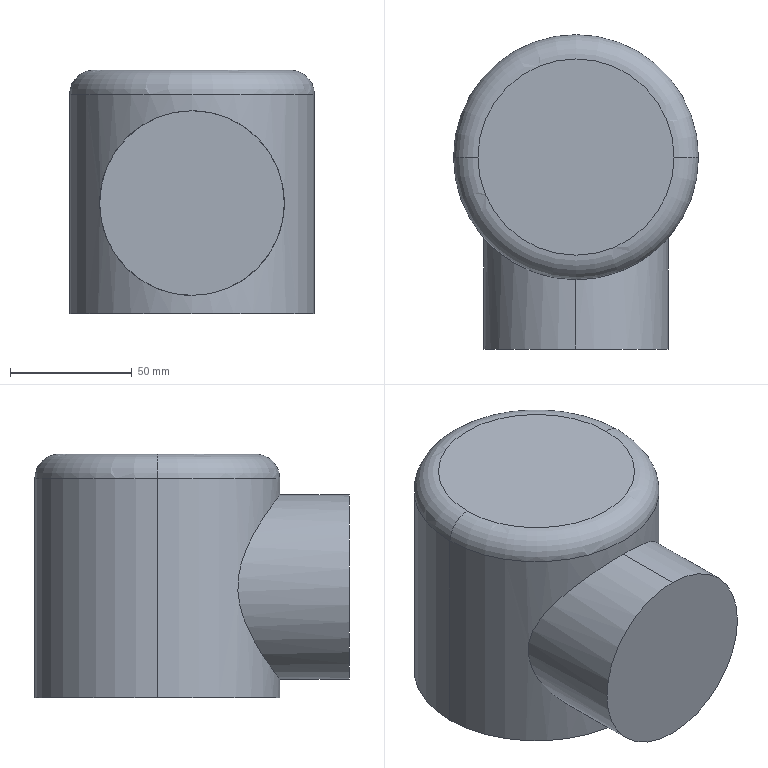Component | SolidWorks | RehabilitationChair-18-3-2 | 1 solid | 9 faces | box 100.49 x 128.95 x 100 mm | volume 932353 mm3 | cylinder 4 | plane 3 | torus 2 | commonest cylinder face diameters 75.746 x2 100.487 x2
STEP:
#1=COLOUR_RGB('',0.7922,0.8196,0.9333);
#2=FILL_AREA_STYLE_COLOUR('',#1);
#3=FILL_AREA_STYLE('',(#2));
#4=SURFACE_STYLE_FILL_AREA(#3);
#5=SURFACE_SIDE_STYLE('',(#4));
#6=SURFACE_STYLE_USAGE(.BOTH.,#5);
#7=PRESENTATION_STYLE_ASSIGNMENT((#6));
#8=CARTESIAN_POINT('',(-6.121,17.859,6.194));
#9=VERTEX_POINT('',#8);
#10=CARTESIAN_POINT('',(-6.121,17.859,3.212));
#11=VERTEX_POINT('',#10);
#12=CARTESIAN_POINT('',(-6.121,17.859,6.194));
#13=CARTESIAN_POINT('',(-6.224,17.859,6.194));
#14=CARTESIAN_POINT('',(-6.325,17.867,6.184));
#15=CARTESIAN_POINT('',(-6.449,17.886,6.158));
#16=CARTESIAN_POINT('',(-6.473,17.89,6.152));
#17=CARTESIAN_POINT('',(-6.522,17.9,6.139));
#18=CARTESIAN_POINT('',(-6.547,17.905,6.132));
#19=CARTESIAN_POINT('',(-6.619,17.922,6.11));
#20=CARTESIAN_POINT('',(-6.665,17.935,6.092));
#21=CARTESIAN_POINT('',(-6.755,17.963,6.053));
#22=CARTESIAN_POINT('',(-6.799,17.978,6.032));
#23=CARTESIAN_POINT('',(-6.863,18.003,5.997));
#24=CARTESIAN_POINT('',(-6.884,18.012,5.985));
#25=CARTESIAN_POINT('',(-6.925,18.029,5.959));
#26=CARTESIAN_POINT('',(-6.945,18.039,5.946));
#27=CARTESIAN_POINT('',(-7.044,18.085,5.878));
#28=CARTESIAN_POINT('',(-7.116,18.125,5.818));
#29=CARTESIAN_POINT('',(-7.198,18.178,5.735));
#30=CARTESIAN_POINT('',(-7.214,18.188,5.718));
#31=CARTESIAN_POINT('',(-7.245,18.209,5.683));
#32=CARTESIAN_POINT('',(-7.261,18.22,5.665));
#33=CARTESIAN_POINT('',(-7.305,18.252,5.611));
#34=CARTESIAN_POINT('',(-7.333,18.273,5.573));
#35=CARTESIAN_POINT('',(-7.41,18.336,5.457));
#36=CARTESIAN_POINT('',(-7.455,18.376,5.375));
#37=CARTESIAN_POINT('',(-7.512,18.43,5.243));
#38=CARTESIAN_POINT('',(-7.529,18.447,5.197));
#39=CARTESIAN_POINT('',(-7.558,18.478,5.103));
#40=CARTESIAN_POINT('',(-7.571,18.491,5.055));
#41=CARTESIAN_POINT('',(-7.586,18.508,4.982));
#42=CARTESIAN_POINT('',(-7.59,18.513,4.957));
#43=CARTESIAN_POINT('',(-7.598,18.521,4.907));
#44=CARTESIAN_POINT('',(-7.601,18.525,4.882));
#45=CARTESIAN_POINT('',(-7.609,18.534,4.805));
#46=CARTESIAN_POINT('',(-7.612,18.537,4.754));
#47=CARTESIAN_POINT('',(-7.612,18.537,4.652));
#48=CARTESIAN_POINT('',(-7.609,18.534,4.601));
#49=CARTESIAN_POINT('',(-7.601,18.525,4.525));
#50=CARTESIAN_POINT('',(-7.598,18.522,4.5));
#51=CARTESIAN_POINT('',(-7.59,18.513,4.45));
#52=CARTESIAN_POINT('',(-7.586,18.508,4.425));
#53=CARTESIAN_POINT('',(-7.571,18.491,4.351));
#54=CARTESIAN_POINT('',(-7.558,18.478,4.303));
#55=CARTESIAN_POINT('',(-7.529,18.447,4.209));
#56=CARTESIAN_POINT('',(-7.512,18.43,4.164));
#57=CARTESIAN_POINT('',(-7.455,18.376,4.031));
#58=CARTESIAN_POINT('',(-7.41,18.335,3.949));
#59=CARTESIAN_POINT('',(-7.332,18.273,3.833));
#60=CARTESIAN_POINT('',(-7.304,18.252,3.795));
#61=CARTESIAN_POINT('',(-7.26,18.22,3.741));
#62=CARTESIAN_POINT('',(-7.244,18.209,3.723));
#63=CARTESIAN_POINT('',(-7.213,18.188,3.688));
#64=CARTESIAN_POINT('',(-7.197,18.177,3.671));
#65=CARTESIAN_POINT('',(-7.115,18.125,3.588));
#66=CARTESIAN_POINT('',(-7.043,18.085,3.528));
#67=CARTESIAN_POINT('',(-6.945,18.039,3.46));
#68=CARTESIAN_POINT('',(-6.925,18.03,3.447));
#69=CARTESIAN_POINT('',(-6.884,18.012,3.422));
#70=CARTESIAN_POINT('',(-6.863,18.003,3.41));
#71=CARTESIAN_POINT('',(-6.799,17.978,3.374));
#72=CARTESIAN_POINT('',(-6.755,17.963,3.353));
#73=CARTESIAN_POINT('',(-6.665,17.934,3.314));
#74=CARTESIAN_POINT('',(-6.618,17.922,3.297));
#75=CARTESIAN_POINT('',(-6.547,17.905,3.274));
#76=CARTESIAN_POINT('',(-6.523,17.9,3.267));
#77=CARTESIAN_POINT('',(-6.474,17.89,3.254));
#78=CARTESIAN_POINT('',(-6.449,17.886,3.248));
#79=CARTESIAN_POINT('',(-6.324,17.867,3.223));
#80=CARTESIAN_POINT('',(-6.223,17.859,3.212));
#81=CARTESIAN_POINT('',(-6.121,17.859,3.212));
#82=B_SPLINE_CURVE_WITH_KNOTS('',3,(#12,#13,#14,#15,#16,#17,#18,#19,#20,#21,#22,#23,#24,#25,#26,#27,#28,#29,#30,#31,#32,#33,#34,#35,#36,#37,#38,#39,#40,#41,#42,#43,#44,#45,#46,#47,#48,#49,#50,#51,#52,#53,#54,#55,#56,#57,#58,#59,#60,#61,#62,#63,#64,#65,#66,#67,#68,#69,#70,#71,#72,#73,#74,#75,#76,#77,#78,#79,#80,#81),.UNSPECIFIED.,.F.,.F.,(4,2,2,2,2,2,2,2,2,2,2,2,2,2,2,2,2,2,2,2,2,2,2,2,2,2,2,2,2,2,2,2,2,2,4),(0.,0.007758,0.009698,0.01164,0.01552,0.0194,0.02134,0.02327,0.03103,0.03297,0.03491,0.03879,0.04655,0.05043,0.05431,0.05625,0.05819,0.06207,0.06594,0.06788,0.06982,0.0737,0.07758,0.08534,0.08922,0.09116,0.0931,0.1009,0.1028,0.1047,0.1086,0.1125,0.1144,0.1164,0.1241),.UNSPECIFIED.);
#83=EDGE_CURVE('',#9,#11,#82,.T.);
#84=ORIENTED_EDGE('',*,*,#83,.T.);
#85=CARTESIAN_POINT('',(-6.121,16.738,3.212));
#86=VERTEX_POINT('',#85);
#87=CARTESIAN_POINT('',(-6.121,20.675,3.212));
#88=DIRECTION('',(0.00000048,-1.,-0.00000005));
#89=VECTOR('',#88,39.37);
#90=LINE('',#87,#89);
#91=EDGE_CURVE('',#11,#86,#90,.T.);
#92=ORIENTED_EDGE('',*,*,#91,.T.);
#93=CARTESIAN_POINT('',(-6.121,16.738,6.194));
#94=VERTEX_POINT('',#93);
#95=CARTESIAN_POINT('',(-6.121,16.738,4.703));
#96=DIRECTION('',(-0.00000048,1.,0.00000005));
#97=DIRECTION('',(0.00000157,0.00000005,-1.));
#98=AXIS2_PLACEMENT_3D('',#95,#96,#97);
#99=CIRCLE('',#98,1.491);
#100=EDGE_CURVE('',#86,#94,#99,.T.);
#101=ORIENTED_EDGE('',*,*,#100,.T.);
#102=CARTESIAN_POINT('',(-6.121,20.675,6.194));
#103=DIRECTION('',(0.00000048,-1.,-0.00000005));
#104=VECTOR('',#103,39.37);
#105=LINE('',#102,#104);
#106=EDGE_CURVE('',#9,#94,#105,.T.);
#107=ORIENTED_EDGE('',*,*,#106,.F.);
#108=EDGE_LOOP('',(#84,#92,#101,#107));
#109=FACE_OUTER_BOUND('',#108,.T.);
#110=CARTESIAN_POINT('',(-6.121,20.675,4.703));
#111=DIRECTION('',(0.00000048,-1.,-0.00000005));
#112=DIRECTION('',(-0.00000157,-0.00000005,1.));
#113=AXIS2_PLACEMENT_3D('',#110,#111,#112);
#114=CYLINDRICAL_SURFACE('',#113,1.491);
#115=ADVANCED_FACE('',(#109),#114,.T.);
#116=CARTESIAN_POINT('',(-8.099,19.837,6.457));
#117=VERTEX_POINT('',#116);
#118=CARTESIAN_POINT('',(-4.143,19.837,6.457));
#119=VERTEX_POINT('',#118);
#120=CARTESIAN_POINT('',(-6.121,19.837,6.457));
#121=DIRECTION('',(0.00000157,0.00000005,-1.));
#122=DIRECTION('',(1.,0.00000048,0.00000157));
#123=AXIS2_PLACEMENT_3D('',#120,#121,#122);
#124=CIRCLE('',#123,1.978);
#125=EDGE_CURVE('',#117,#119,#124,.T.);
#126=ORIENTED_EDGE('',*,*,#125,.F.);
#127=CARTESIAN_POINT('',(-7.705,19.837,6.85));
#128=VERTEX_POINT('',#127);
#129=CARTESIAN_POINT('',(-7.705,19.837,6.457));
#130=DIRECTION('',(-0.00000048,1.,0.00000005));
#131=DIRECTION('',(-1.,-0.00000048,0.));
#132=AXIS2_PLACEMENT_3D('',#129,#130,#131);
#133=CIRCLE('',#132,0.3937);
#134=EDGE_CURVE('',#117,#128,#133,.T.);
#135=ORIENTED_EDGE('',*,*,#134,.T.);
#136=CARTESIAN_POINT('',(-4.536,19.837,6.85));
#137=VERTEX_POINT('',#136);
#138=CARTESIAN_POINT('',(-6.121,19.837,6.85));
#139=DIRECTION('',(-0.00000157,-0.00000005,1.));
#140=DIRECTION('',(1.,0.00000048,0.00000157));
#141=AXIS2_PLACEMENT_3D('',#138,#139,#140);
#142=CIRCLE('',#141,1.584);
#143=EDGE_CURVE('',#137,#128,#142,.T.);
#144=ORIENTED_EDGE('',*,*,#143,.F.);
#145=CARTESIAN_POINT('',(-4.536,19.837,6.457));
#146=DIRECTION('',(0.00000048,-1.,-0.00000005));
#147=DIRECTION('',(1.,0.00000048,0.));
#148=AXIS2_PLACEMENT_3D('',#145,#146,#147);
#149=CIRCLE('',#148,0.3937);
#150=EDGE_CURVE('',#119,#137,#149,.T.);
#151=ORIENTED_EDGE('',*,*,#150,.F.);
#152=EDGE_LOOP('',(#126,#135,#144,#151));
#153=FACE_OUTER_BOUND('',#152,.T.);
#154=CARTESIAN_POINT('',(-6.121,19.837,6.457));
#155=DIRECTION('',(-0.00000157,-0.00000005,1.));
#156=DIRECTION('',(1.,0.00000048,0.00000157));
#157=AXIS2_PLACEMENT_3D('',#154,#155,#156);
#158=TOROIDAL_SURFACE('',#157,1.584,0.3937);
#159=ADVANCED_FACE('',(#153),#158,.T.);
#160=ORIENTED_EDGE('',*,*,#125,.T.);
#161=CARTESIAN_POINT('',(-4.143,19.837,2.913));
#162=VERTEX_POINT('',#161);
#163=CARTESIAN_POINT('',(-4.143,19.837,6.85));
#164=DIRECTION('',(0.00000157,0.00000005,-1.));
#165=VECTOR('',#164,39.37);
#166=LINE('',#163,#165);
#167=EDGE_CURVE('',#119,#162,#166,.T.);
#168=ORIENTED_EDGE('',*,*,#167,.T.);
#169=CARTESIAN_POINT('',(-8.099,19.837,2.913));
#170=VERTEX_POINT('',#169);
#171=CARTESIAN_POINT('',(-6.121,19.837,2.913));
#172=DIRECTION('',(-0.00000157,-0.00000005,1.));
#173=DIRECTION('',(1.,0.00000048,0.00000157));
#174=AXIS2_PLACEMENT_3D('',#171,#172,#173);
#175=CIRCLE('',#174,1.978);
#176=EDGE_CURVE('',#162,#170,#175,.T.);
#177=ORIENTED_EDGE('',*,*,#176,.T.);
#178=CARTESIAN_POINT('',(-8.099,19.837,6.85));
#179=DIRECTION('',(0.00000157,0.00000005,-1.));
#180=VECTOR('',#179,39.37);
#181=LINE('',#178,#180);
#182=EDGE_CURVE('',#117,#170,#181,.T.);
#183=ORIENTED_EDGE('',*,*,#182,.F.);
#184=EDGE_LOOP('',(#160,#168,#177,#183));
#185=FACE_OUTER_BOUND('',#184,.T.);
#186=CARTESIAN_POINT('',(-6.121,19.837,6.85));
#187=DIRECTION('',(0.00000157,0.00000005,-1.));
#188=DIRECTION('',(-1.,-0.00000048,-0.00000157));
#189=AXIS2_PLACEMENT_3D('',#186,#187,#188);
#190=CYLINDRICAL_SURFACE('',#189,1.978);
#191=ADVANCED_FACE('',(#185),#190,.T.);
#192=ORIENTED_EDGE('',*,*,#167,.F.);
#193=CARTESIAN_POINT('',(-6.121,19.837,6.457));
#194=DIRECTION('',(0.00000157,0.00000005,-1.));
#195=DIRECTION('',(1.,0.00000048,0.00000157));
#196=AXIS2_PLACEMENT_3D('',#193,#194,#195);
#197=CIRCLE('',#196,1.978);
#198=EDGE_CURVE('',#119,#117,#197,.T.);
#199=ORIENTED_EDGE('',*,*,#198,.T.);
#200=ORIENTED_EDGE('',*,*,#182,.T.);
#201=CARTESIAN_POINT('',(-6.121,19.837,2.913));
#202=DIRECTION('',(-0.00000157,-0.00000005,1.));
#203=DIRECTION('',(1.,0.00000048,0.00000157));
#204=AXIS2_PLACEMENT_3D('',#201,#202,#203);
#205=CIRCLE('',#204,1.978);
#206=EDGE_CURVE('',#170,#162,#205,.T.);
#207=ORIENTED_EDGE('',*,*,#206,.T.);
#208=EDGE_LOOP('',(#192,#199,#200,#207));
#209=FACE_OUTER_BOUND('',#208,.T.);
#210=ORIENTED_EDGE('',*,*,#83,.F.);
#211=CARTESIAN_POINT('',(-6.121,17.859,3.212));
#212=CARTESIAN_POINT('',(-6.095,17.859,3.212));
#213=CARTESIAN_POINT('',(-6.07,17.859,3.213));
#214=CARTESIAN_POINT('',(-6.018,17.861,3.215));
#215=CARTESIAN_POINT('',(-5.993,17.863,3.217));
#216=CARTESIAN_POINT('',(-5.916,17.869,3.225));
#217=CARTESIAN_POINT('',(-5.866,17.875,3.233));
#218=CARTESIAN_POINT('',(-5.767,17.89,3.254));
#219=CARTESIAN_POINT('',(-5.719,17.9,3.267));
#220=CARTESIAN_POINT('',(-5.647,17.916,3.289));
#221=CARTESIAN_POINT('',(-5.623,17.922,3.297));
#222=CARTESIAN_POINT('',(-5.576,17.935,3.315));
#223=CARTESIAN_POINT('',(-5.553,17.942,3.324));
#224=CARTESIAN_POINT('',(-5.44,17.977,3.373));
#225=CARTESIAN_POINT('',(-5.356,18.011,3.42));
#226=CARTESIAN_POINT('',(-5.257,18.057,3.488));
#227=CARTESIAN_POINT('',(-5.237,18.067,3.502));
#228=CARTESIAN_POINT('',(-5.2,18.086,3.531));
#229=CARTESIAN_POINT('',(-5.181,18.096,3.545));
#230=CARTESIAN_POINT('',(-5.127,18.126,3.591));
#231=CARTESIAN_POINT('',(-5.093,18.147,3.622));
#232=CARTESIAN_POINT('',(-5.027,18.188,3.689));
#233=CARTESIAN_POINT('',(-4.996,18.209,3.723));
#234=CARTESIAN_POINT('',(-4.951,18.241,3.778));
#235=CARTESIAN_POINT('',(-4.937,18.252,3.796));
#236=CARTESIAN_POINT('',(-4.909,18.273,3.834));
#237=CARTESIAN_POINT('',(-4.896,18.284,3.853));
#238=CARTESIAN_POINT('',(-4.831,18.336,3.95));
#239=CARTESIAN_POINT('',(-4.786,18.376,4.032));
#240=CARTESIAN_POINT('',(-4.73,18.43,4.163));
#241=CARTESIAN_POINT('',(-4.713,18.447,4.209));
#242=CARTESIAN_POINT('',(-4.691,18.47,4.279));
#243=CARTESIAN_POINT('',(-4.684,18.477,4.303));
#244=CARTESIAN_POINT('',(-4.672,18.491,4.351));
#245=CARTESIAN_POINT('',(-4.666,18.497,4.375));
#246=CARTESIAN_POINT('',(-4.651,18.513,4.449));
#247=CARTESIAN_POINT('',(-4.643,18.522,4.499));
#248=CARTESIAN_POINT('',(-4.635,18.531,4.575));
#249=CARTESIAN_POINT('',(-4.633,18.533,4.601));
#250=CARTESIAN_POINT('',(-4.63,18.536,4.652));
#251=CARTESIAN_POINT('',(-4.63,18.537,4.678));
#252=CARTESIAN_POINT('',(-4.63,18.537,4.755));
#253=CARTESIAN_POINT('',(-4.632,18.534,4.806));
#254=CARTESIAN_POINT('',(-4.64,18.525,4.881));
#255=CARTESIAN_POINT('',(-4.643,18.522,4.907));
#256=CARTESIAN_POINT('',(-4.651,18.513,4.957));
#257=CARTESIAN_POINT('',(-4.656,18.508,4.982));
#258=CARTESIAN_POINT('',(-4.671,18.491,5.056));
#259=CARTESIAN_POINT('',(-4.684,18.478,5.104));
#260=CARTESIAN_POINT('',(-4.713,18.447,5.197));
#261=CARTESIAN_POINT('',(-4.73,18.43,5.242));
#262=CARTESIAN_POINT('',(-4.767,18.394,5.33));
#263=CARTESIAN_POINT('',(-4.788,18.375,5.374));
#264=CARTESIAN_POINT('',(-4.833,18.335,5.457));
#265=CARTESIAN_POINT('',(-4.857,18.314,5.497));
#266=CARTESIAN_POINT('',(-4.935,18.252,5.612));
#267=CARTESIAN_POINT('',(-4.994,18.209,5.684));
#268=CARTESIAN_POINT('',(-5.093,18.147,5.784));
#269=CARTESIAN_POINT('',(-5.128,18.126,5.816));
#270=CARTESIAN_POINT('',(-5.2,18.086,5.877));
#271=CARTESIAN_POINT('',(-5.237,18.067,5.905));
#272=CARTESIAN_POINT('',(-5.354,18.011,5.986));
#273=CARTESIAN_POINT('',(-5.438,17.978,6.033));
#274=CARTESIAN_POINT('',(-5.552,17.942,6.082));
#275=CARTESIAN_POINT('',(-5.575,17.936,6.091));
#276=CARTESIAN_POINT('',(-5.622,17.923,6.108));
#277=CARTESIAN_POINT('',(-5.645,17.917,6.117));
#278=CARTESIAN_POINT('',(-5.717,17.9,6.139));
#279=CARTESIAN_POINT('',(-5.765,17.89,6.152));
#280=CARTESIAN_POINT('',(-5.864,17.875,6.173));
#281=CARTESIAN_POINT('',(-5.915,17.869,6.181));
#282=CARTESIAN_POINT('',(-5.992,17.863,6.189));
#283=CARTESIAN_POINT('',(-6.017,17.861,6.191));
#284=CARTESIAN_POINT('',(-6.056,17.86,6.193));
#285=CARTESIAN_POINT('',(-6.069,17.859,6.193));
#286=CARTESIAN_POINT('',(-6.095,17.859,6.194));
#287=CARTESIAN_POINT('',(-6.108,17.859,6.194));
#288=CARTESIAN_POINT('',(-6.121,17.859,6.194));
#289=B_SPLINE_CURVE_WITH_KNOTS('',3,(#211,#212,#213,#214,#215,#216,#217,#218,#219,#220,#221,#222,#223,#224,#225,#226,#227,#228,#229,#230,#231,#232,#233,#234,#235,#236,#237,#238,#239,#240,#241,#242,#243,#244,#245,#246,#247,#248,#249,#250,#251,#252,#253,#254,#255,#256,#257,#258,#259,#260,#261,#262,#263,#264,#265,#266,#267,#268,#269,#270,#271,#272,#273,#274,#275,#276,#277,#278,#279,#280,#281,#282,#283,#284,#285,#286,#287,#288),.UNSPECIFIED.,.F.,.F.,(4,2,2,2,2,2,2,2,2,2,2,2,2,2,2,2,2,2,2,2,2,2,2,2,2,2,2,2,2,2,2,2,2,2,2,2,2,2,4),(0.1241,0.1261,0.128,0.1319,0.1357,0.1377,0.1396,0.1474,0.1493,0.1512,0.1551,0.159,0.1609,0.1628,0.1706,0.1745,0.1764,0.1783,0.1822,0.1841,0.1861,0.1899,0.1919,0.1938,0.1977,0.2016,0.2054,0.2093,0.217,0.2209,0.2248,0.2325,0.2345,0.2364,0.2403,0.2441,0.2461,0.247,0.248),.UNSPECIFIED.);
#290=EDGE_CURVE('',#11,#9,#289,.T.);
#291=ORIENTED_EDGE('',*,*,#290,.F.);
#292=EDGE_LOOP('',(#210,#291));
#293=FACE_BOUND('',#292,.T.);
#294=CARTESIAN_POINT('',(-6.121,19.837,6.85));
#295=DIRECTION('',(0.00000157,0.00000005,-1.));
#296=DIRECTION('',(-1.,-0.00000048,-0.00000157));
#297=AXIS2_PLACEMENT_3D('',#294,#295,#296);
#298=CYLINDRICAL_SURFACE('',#297,1.978);
#299=ADVANCED_FACE('',(#209,#293),#298,.T.);
#300=ORIENTED_EDGE('',*,*,#143,.T.);
#301=CARTESIAN_POINT('',(-6.121,19.837,6.85));
#302=DIRECTION('',(-0.00000157,-0.00000005,1.));
#303=DIRECTION('',(1.,0.00000048,0.00000157));
#304=AXIS2_PLACEMENT_3D('',#301,#302,#303);
#305=CIRCLE('',#304,1.584);
#306=EDGE_CURVE('',#128,#137,#305,.T.);
#307=ORIENTED_EDGE('',*,*,#306,.T.);
#308=EDGE_LOOP('',(#300,#307));
#309=FACE_OUTER_BOUND('',#308,.T.);
#310=CARTESIAN_POINT('',(-6.121,19.837,6.85));
#311=DIRECTION('',(-0.00000157,-0.00000005,1.));
#312=DIRECTION('',(1.,0.00000048,0.00000157));
#313=AXIS2_PLACEMENT_3D('',#310,#311,#312);
#314=PLANE('',#313);
#315=ADVANCED_FACE('',(#309),#314,.T.);
#316=ORIENTED_EDGE('',*,*,#134,.F.);
#317=ORIENTED_EDGE('',*,*,#198,.F.);
#318=ORIENTED_EDGE('',*,*,#150,.T.);
#319=ORIENTED_EDGE('',*,*,#306,.F.);
#320=EDGE_LOOP('',(#316,#317,#318,#319));
#321=FACE_OUTER_BOUND('',#320,.T.);
#322=CARTESIAN_POINT('',(-6.121,19.837,6.457));
#323=DIRECTION('',(-0.00000157,-0.00000005,1.));
#324=DIRECTION('',(1.,0.00000048,0.00000157));
#325=AXIS2_PLACEMENT_3D('',#322,#323,#324);
#326=TOROIDAL_SURFACE('',#325,1.584,0.3937);
#327=ADVANCED_FACE('',(#321),#326,.T.);
#328=ORIENTED_EDGE('',*,*,#91,.F.);
#329=ORIENTED_EDGE('',*,*,#290,.T.);
#330=ORIENTED_EDGE('',*,*,#106,.T.);
#331=CARTESIAN_POINT('',(-6.121,16.738,4.703));
#332=DIRECTION('',(-0.00000048,1.,0.00000005));
#333=DIRECTION('',(0.00000157,0.00000005,-1.));
#334=AXIS2_PLACEMENT_3D('',#331,#332,#333);
#335=CIRCLE('',#334,1.491);
#336=EDGE_CURVE('',#94,#86,#335,.T.);
#337=ORIENTED_EDGE('',*,*,#336,.T.);
#338=EDGE_LOOP('',(#328,#329,#330,#337));
#339=FACE_OUTER_BOUND('',#338,.T.);
#340=CARTESIAN_POINT('',(-6.121,20.675,4.703));
#341=DIRECTION('',(0.00000048,-1.,-0.00000005));
#342=DIRECTION('',(-0.00000157,-0.00000005,1.));
#343=AXIS2_PLACEMENT_3D('',#340,#341,#342);
#344=CYLINDRICAL_SURFACE('',#343,1.491);
#345=ADVANCED_FACE('',(#339),#344,.T.);
#346=ORIENTED_EDGE('',*,*,#336,.F.);
#347=ORIENTED_EDGE('',*,*,#100,.F.);
#348=EDGE_LOOP('',(#346,#347));
#349=FACE_OUTER_BOUND('',#348,.T.);
#350=CARTESIAN_POINT('',(-12.242,16.738,-0.00000972));
#351=DIRECTION('',(-0.00000048,1.,0.00000005));
#352=DIRECTION('',(0.00000157,0.00000005,-1.));
#353=AXIS2_PLACEMENT_3D('',#350,#351,#352);
#354=PLANE('',#353);
#355=ADVANCED_FACE('',(#349),#354,.F.);
#356=ORIENTED_EDGE('',*,*,#206,.F.);
#357=ORIENTED_EDGE('',*,*,#176,.F.);
#358=EDGE_LOOP('',(#356,#357));
#359=FACE_OUTER_BOUND('',#358,.T.);
#360=CARTESIAN_POINT('',(-12.242,-0.00000279,2.913));
#361=DIRECTION('',(-0.00000157,-0.00000005,1.));
#362=DIRECTION('',(1.,0.00000048,0.00000157));
#363=AXIS2_PLACEMENT_3D('',#360,#361,#362);
#364=PLANE('',#363);
#365=ADVANCED_FACE('',(#359),#364,.F.);
#366=CLOSED_SHELL('',(#115,#159,#191,#299,#315,#327,#345,#355,#365));
#367=MANIFOLD_SOLID_BREP('',#366);
#368=STYLED_ITEM('',(#7),#367);
#369=(LENGTH_UNIT()NAMED_UNIT(*)SI_UNIT($,.METRE.));
#370=LENGTH_MEASURE_WITH_UNIT(LENGTH_MEASURE(0.0254),#369);
#371=DIMENSIONAL_EXPONENTS(1.,0.,0.,0.,0.,0.,0.);
#372=(CONVERSION_BASED_UNIT('',#370)LENGTH_UNIT()NAMED_UNIT(#371));
#373=UNCERTAINTY_MEASURE_WITH_UNIT(LENGTH_MEASURE(0.00001),#372,'','');
#374=(NAMED_UNIT(*)PLANE_ANGLE_UNIT()SI_UNIT($,.RADIAN.));
#375=(NAMED_UNIT(*)SI_UNIT($,.STERADIAN.)SOLID_ANGLE_UNIT());
#376=(GEOMETRIC_REPRESENTATION_CONTEXT(3)GLOBAL_UNCERTAINTY_ASSIGNED_CONTEXT((#373))GLOBAL_UNIT_ASSIGNED_CONTEXT((#372,#374,#375))REPRESENTATION_CONTEXT('',''));
#377=MECHANICAL_DESIGN_GEOMETRIC_PRESENTATION_REPRESENTATION('',(#368),#376);
#378=PRESENTATION_LAYER_ASSIGNMENT('','',(#368));
#379=CARTESIAN_POINT('',(0.,0.,0.));
#380=DIRECTION('',(0.,0.,1.));
#381=DIRECTION('',(1.,0.,0.));
#382=AXIS2_PLACEMENT_3D('',#379,#380,#381);
#383=(LENGTH_UNIT()NAMED_UNIT(*)SI_UNIT($,.METRE.));
#384=LENGTH_MEASURE_WITH_UNIT(LENGTH_MEASURE(0.0254),#383);
#385=DIMENSIONAL_EXPONENTS(1.,0.,0.,0.,0.,0.,0.);
#386=(CONVERSION_BASED_UNIT('',#384)LENGTH_UNIT()NAMED_UNIT(#385));
#387=UNCERTAINTY_MEASURE_WITH_UNIT(LENGTH_MEASURE(0.00001),#386,'','');
#388=(NAMED_UNIT(*)PLANE_ANGLE_UNIT()SI_UNIT($,.RADIAN.));
#389=(NAMED_UNIT(*)SI_UNIT($,.STERADIAN.)SOLID_ANGLE_UNIT());
#390=(GEOMETRIC_REPRESENTATION_CONTEXT(3)GLOBAL_UNCERTAINTY_ASSIGNED_CONTEXT((#387))GLOBAL_UNIT_ASSIGNED_CONTEXT((#386,#388,#389))REPRESENTATION_CONTEXT('',''));
#391=ADVANCED_BREP_SHAPE_REPRESENTATION('',(#367,#382),#390);